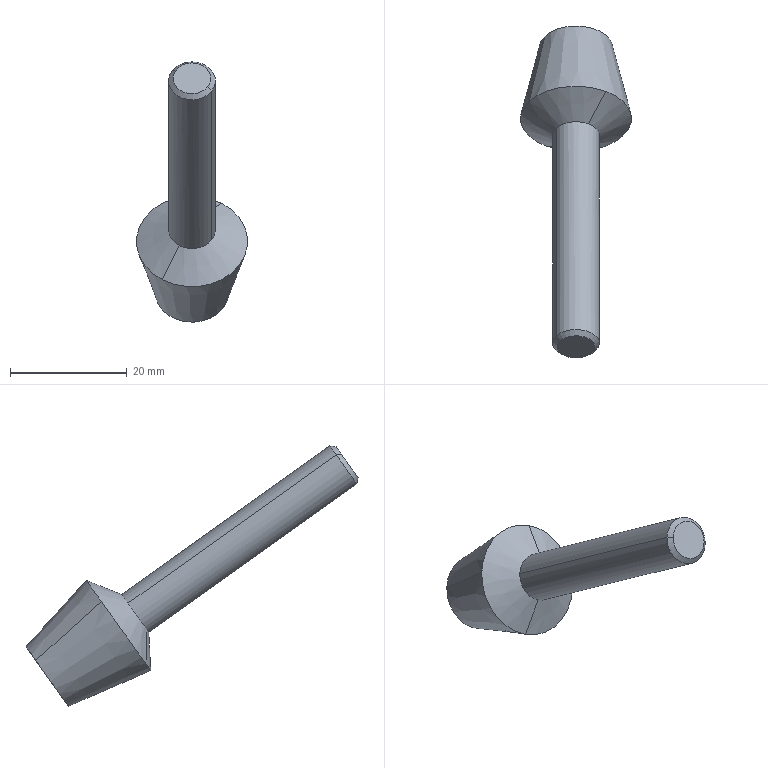Component | SolidWorks | AD12-MC01H-4_2_03.SDASM-1_AD12-_MC01H-4_bo.sdprt-1 | 1 solid | 10 faces | box 19 x 56.78 x 44.52 mm | volume 5722 mm3 | cone 6 | cylinder 2 | plane 2 | commonest cylinder face diameters 8 x2
STEP:
#1=COLOUR_RGB('',0.7922,0.8196,0.9333);
#2=FILL_AREA_STYLE_COLOUR('',#1);
#3=FILL_AREA_STYLE('',(#2));
#4=SURFACE_STYLE_FILL_AREA(#3);
#5=SURFACE_SIDE_STYLE('',(#4));
#6=SURFACE_STYLE_USAGE(.BOTH.,#5);
#7=PRESENTATION_STYLE_ASSIGNMENT((#6));
#8=CARTESIAN_POINT('',(-12.196,-6.944,14.752));
#9=VERTEX_POINT('',#8);
#10=CARTESIAN_POINT('',(-12.413,-6.972,14.713));
#11=VERTEX_POINT('',#10);
#12=CARTESIAN_POINT('',(-12.28,-7.021,14.644));
#13=DIRECTION('',(0.,-0.8137,0.5813));
#14=DIRECTION('',(0.8451,-0.3107,-0.435));
#15=AXIS2_PLACEMENT_3D('',#12,#13,#14);
#16=CIRCLE('',#15,0.1575);
#17=EDGE_CURVE('',#9,#11,#16,.T.);
#18=ORIENTED_EDGE('',*,*,#17,.T.);
#19=CARTESIAN_POINT('',(-12.413,-8.373,15.714));
#20=VERTEX_POINT('',#19);
#21=CARTESIAN_POINT('',(-12.413,-6.38,14.289));
#22=DIRECTION('',(0.,-0.8137,0.5813));
#23=VECTOR('',#22,39.37);
#24=LINE('',#21,#23);
#25=EDGE_CURVE('',#11,#20,#24,.T.);
#26=ORIENTED_EDGE('',*,*,#25,.T.);
#27=CARTESIAN_POINT('',(-12.147,-8.471,15.577));
#28=VERTEX_POINT('',#27);
#29=CARTESIAN_POINT('',(-12.28,-8.422,15.645));
#30=DIRECTION('',(-0.,0.8137,-0.5813));
#31=DIRECTION('',(0.8451,-0.3107,-0.435));
#32=AXIS2_PLACEMENT_3D('',#29,#30,#31);
#33=CIRCLE('',#32,0.1575);
#34=EDGE_CURVE('',#20,#28,#33,.T.);
#35=ORIENTED_EDGE('',*,*,#34,.T.);
#36=CARTESIAN_POINT('',(-12.147,-7.07,14.576));
#37=VERTEX_POINT('',#36);
#38=CARTESIAN_POINT('',(-12.147,-6.478,14.152));
#39=DIRECTION('',(0.,-0.8137,0.5813));
#40=VECTOR('',#39,39.37);
#41=LINE('',#38,#40);
#42=EDGE_CURVE('',#37,#28,#41,.T.);
#43=ORIENTED_EDGE('',*,*,#42,.F.);
#44=CARTESIAN_POINT('',(-12.28,-7.021,14.644));
#45=DIRECTION('',(0.,-0.8137,0.5813));
#46=DIRECTION('',(0.8451,-0.3107,-0.435));
#47=AXIS2_PLACEMENT_3D('',#44,#45,#46);
#48=CIRCLE('',#47,0.1575);
#49=EDGE_CURVE('',#37,#9,#48,.T.);
#50=ORIENTED_EDGE('',*,*,#49,.T.);
#51=EDGE_LOOP('',(#18,#26,#35,#43,#50));
#52=FACE_OUTER_BOUND('',#51,.T.);
#53=CARTESIAN_POINT('',(-12.28,-6.429,14.221));
#54=DIRECTION('',(0.,-0.8137,0.5813));
#55=DIRECTION('',(0.8451,-0.3107,-0.435));
#56=AXIS2_PLACEMENT_3D('',#53,#54,#55);
#57=CYLINDRICAL_SURFACE('',#56,0.1575);
#58=ADVANCED_FACE('',(#52),#57,.T.);
#59=CARTESIAN_POINT('',(-12.388,-8.407,15.718));
#60=VERTEX_POINT('',#59);
#61=CARTESIAN_POINT('',(-12.173,-8.486,15.607));
#62=VERTEX_POINT('',#61);
#63=CARTESIAN_POINT('',(-12.28,-8.447,15.663));
#64=DIRECTION('',(-0.,0.8137,-0.5813));
#65=DIRECTION('',(-0.8451,0.3107,0.435));
#66=AXIS2_PLACEMENT_3D('',#63,#64,#65);
#67=CIRCLE('',#66,0.1273);
#68=EDGE_CURVE('',#60,#62,#67,.T.);
#69=ORIENTED_EDGE('',*,*,#68,.T.);
#70=CARTESIAN_POINT('',(-12.147,-8.471,15.577));
#71=DIRECTION('',(0.5976,0.3556,-0.7186));
#72=VECTOR('',#71,39.37);
#73=LINE('',#70,#72);
#74=EDGE_CURVE('',#62,#28,#73,.T.);
#75=ORIENTED_EDGE('',*,*,#74,.T.);
#76=ORIENTED_EDGE('',*,*,#34,.F.);
#77=CARTESIAN_POINT('',(-12.413,-8.373,15.714));
#78=DIRECTION('',(-0.5976,0.7951,-0.1035));
#79=VECTOR('',#78,39.37);
#80=LINE('',#77,#79);
#81=EDGE_CURVE('',#60,#20,#80,.T.);
#82=ORIENTED_EDGE('',*,*,#81,.F.);
#83=EDGE_LOOP('',(#69,#75,#76,#82));
#84=FACE_OUTER_BOUND('',#83,.T.);
#85=CARTESIAN_POINT('',(-12.28,-8.422,15.645));
#86=DIRECTION('',(-0.,0.8137,-0.5813));
#87=DIRECTION('',(-0.8451,0.3107,0.435));
#88=AXIS2_PLACEMENT_3D('',#85,#86,#87);
#89=CONICAL_SURFACE('',#88,0.1575,0.7854);
#90=ADVANCED_FACE('',(#84),#89,.T.);
#91=CARTESIAN_POINT('',(-12.364,-7.099,14.536));
#92=VERTEX_POINT('',#91);
#93=CARTESIAN_POINT('',(-12.28,-7.021,14.644));
#94=DIRECTION('',(0.,-0.8137,0.5813));
#95=DIRECTION('',(0.8451,-0.3107,-0.435));
#96=AXIS2_PLACEMENT_3D('',#93,#94,#95);
#97=CIRCLE('',#96,0.1575);
#98=EDGE_CURVE('',#92,#37,#97,.T.);
#99=ORIENTED_EDGE('',*,*,#98,.F.);
#100=CARTESIAN_POINT('',(-12.48,-7.093,14.307));
#101=VERTEX_POINT('',#100);
#102=CARTESIAN_POINT('',(-12.48,-7.093,14.307));
#103=DIRECTION('',(-0.451,0.02239,-0.8922));
#104=VECTOR('',#103,39.37);
#105=LINE('',#102,#104);
#106=EDGE_CURVE('',#92,#101,#105,.T.);
#107=ORIENTED_EDGE('',*,*,#106,.T.);
#108=CARTESIAN_POINT('',(-11.964,-7.025,14.401));
#109=VERTEX_POINT('',#108);
#110=CARTESIAN_POINT('',(-12.28,-6.909,14.564));
#111=DIRECTION('',(0.,-0.8137,0.5813));
#112=DIRECTION('',(-0.8451,0.3107,0.435));
#113=AXIS2_PLACEMENT_3D('',#110,#111,#112);
#114=CIRCLE('',#113,0.374);
#115=EDGE_CURVE('',#101,#109,#114,.T.);
#116=ORIENTED_EDGE('',*,*,#115,.T.);
#117=CARTESIAN_POINT('',(-12.08,-6.725,14.821));
#118=VERTEX_POINT('',#117);
#119=CARTESIAN_POINT('',(-12.28,-6.909,14.564));
#120=DIRECTION('',(0.,-0.8137,0.5813));
#121=DIRECTION('',(-0.8451,0.3107,0.435));
#122=AXIS2_PLACEMENT_3D('',#119,#120,#121);
#123=CIRCLE('',#122,0.374);
#124=EDGE_CURVE('',#109,#118,#123,.T.);
#125=ORIENTED_EDGE('',*,*,#124,.T.);
#126=CARTESIAN_POINT('',(-12.08,-6.725,14.821));
#127=DIRECTION('',(0.451,0.8513,0.2681));
#128=VECTOR('',#127,39.37);
#129=LINE('',#126,#128);
#130=EDGE_CURVE('',#9,#118,#129,.T.);
#131=ORIENTED_EDGE('',*,*,#130,.F.);
#132=ORIENTED_EDGE('',*,*,#49,.F.);
#133=EDGE_LOOP('',(#99,#107,#116,#125,#131,#132));
#134=FACE_OUTER_BOUND('',#133,.T.);
#135=CARTESIAN_POINT('',(-12.28,-6.909,14.564));
#136=DIRECTION('',(0.,0.8137,-0.5813));
#137=DIRECTION('',(0.5346,0.4913,0.6877));
#138=AXIS2_PLACEMENT_3D('',#135,#136,#137);
#139=CONICAL_SURFACE('',#138,0.374,1.004);
#140=ADVANCED_FACE('',(#134),#139,.T.);
#141=CARTESIAN_POINT('',(-12.072,-6.505,14.114));
#142=VERTEX_POINT('',#141);
#143=CARTESIAN_POINT('',(-12.488,-6.352,14.328));
#144=VERTEX_POINT('',#143);
#145=CARTESIAN_POINT('',(-12.28,-6.429,14.221));
#146=DIRECTION('',(0.,-0.8137,0.5813));
#147=DIRECTION('',(0.8451,-0.3107,-0.435));
#148=AXIS2_PLACEMENT_3D('',#145,#146,#147);
#149=CIRCLE('',#148,0.2461);
#150=EDGE_CURVE('',#142,#144,#149,.T.);
#151=ORIENTED_EDGE('',*,*,#150,.T.);
#152=CARTESIAN_POINT('',(-12.596,-6.793,14.727));
#153=VERTEX_POINT('',#152);
#154=CARTESIAN_POINT('',(-12.596,-6.793,14.727));
#155=DIRECTION('',(-0.179,-0.7294,0.6602));
#156=VECTOR('',#155,39.37);
#157=LINE('',#154,#156);
#158=EDGE_CURVE('',#144,#153,#157,.T.);
#159=ORIENTED_EDGE('',*,*,#158,.T.);
#160=CARTESIAN_POINT('',(-12.28,-6.909,14.564));
#161=DIRECTION('',(0.,-0.8137,0.5813));
#162=DIRECTION('',(-0.8451,0.3107,0.435));
#163=AXIS2_PLACEMENT_3D('',#160,#161,#162);
#164=CIRCLE('',#163,0.374);
#165=EDGE_CURVE('',#118,#153,#164,.T.);
#166=ORIENTED_EDGE('',*,*,#165,.F.);
#167=ORIENTED_EDGE('',*,*,#124,.F.);
#168=CARTESIAN_POINT('',(-11.964,-7.025,14.401));
#169=DIRECTION('',(0.179,-0.861,0.476));
#170=VECTOR('',#169,39.37);
#171=LINE('',#168,#170);
#172=EDGE_CURVE('',#142,#109,#171,.T.);
#173=ORIENTED_EDGE('',*,*,#172,.F.);
#174=EDGE_LOOP('',(#151,#159,#166,#167,#173));
#175=FACE_OUTER_BOUND('',#174,.T.);
#176=CARTESIAN_POINT('',(-12.28,-6.909,14.564));
#177=DIRECTION('',(0.,-0.8137,0.5813));
#178=DIRECTION('',(0.8451,-0.3107,-0.435));
#179=AXIS2_PLACEMENT_3D('',#176,#177,#178);
#180=CONICAL_SURFACE('',#179,0.374,0.2134);
#181=ADVANCED_FACE('',(#175),#180,.T.);
#182=ORIENTED_EDGE('',*,*,#25,.F.);
#183=CARTESIAN_POINT('',(-12.28,-7.021,14.644));
#184=DIRECTION('',(0.,-0.8137,0.5813));
#185=DIRECTION('',(0.8451,-0.3107,-0.435));
#186=AXIS2_PLACEMENT_3D('',#183,#184,#185);
#187=CIRCLE('',#186,0.1575);
#188=EDGE_CURVE('',#11,#92,#187,.T.);
#189=ORIENTED_EDGE('',*,*,#188,.T.);
#190=ORIENTED_EDGE('',*,*,#98,.T.);
#191=ORIENTED_EDGE('',*,*,#42,.T.);
#192=CARTESIAN_POINT('',(-12.28,-8.422,15.645));
#193=DIRECTION('',(-0.,0.8137,-0.5813));
#194=DIRECTION('',(0.8451,-0.3107,-0.435));
#195=AXIS2_PLACEMENT_3D('',#192,#193,#194);
#196=CIRCLE('',#195,0.1575);
#197=EDGE_CURVE('',#28,#20,#196,.T.);
#198=ORIENTED_EDGE('',*,*,#197,.T.);
#199=EDGE_LOOP('',(#182,#189,#190,#191,#198));
#200=FACE_OUTER_BOUND('',#199,.T.);
#201=CARTESIAN_POINT('',(-12.28,-6.429,14.221));
#202=DIRECTION('',(0.,-0.8137,0.5813));
#203=DIRECTION('',(0.8451,-0.3107,-0.435));
#204=AXIS2_PLACEMENT_3D('',#201,#202,#203);
#205=CYLINDRICAL_SURFACE('',#204,0.1575);
#206=ADVANCED_FACE('',(#200),#205,.T.);
#207=ORIENTED_EDGE('',*,*,#74,.F.);
#208=CARTESIAN_POINT('',(-12.28,-8.447,15.663));
#209=DIRECTION('',(-0.,0.8137,-0.5813));
#210=DIRECTION('',(-0.8451,0.3107,0.435));
#211=AXIS2_PLACEMENT_3D('',#208,#209,#210);
#212=CIRCLE('',#211,0.1273);
#213=EDGE_CURVE('',#62,#60,#212,.T.);
#214=ORIENTED_EDGE('',*,*,#213,.T.);
#215=ORIENTED_EDGE('',*,*,#81,.T.);
#216=ORIENTED_EDGE('',*,*,#197,.F.);
#217=EDGE_LOOP('',(#207,#214,#215,#216));
#218=FACE_OUTER_BOUND('',#217,.T.);
#219=CARTESIAN_POINT('',(-12.28,-8.422,15.645));
#220=DIRECTION('',(-0.,0.8137,-0.5813));
#221=DIRECTION('',(-0.8451,0.3107,0.435));
#222=AXIS2_PLACEMENT_3D('',#219,#220,#221);
#223=CONICAL_SURFACE('',#222,0.1575,0.7854);
#224=ADVANCED_FACE('',(#218),#223,.T.);
#225=ORIENTED_EDGE('',*,*,#106,.F.);
#226=ORIENTED_EDGE('',*,*,#188,.F.);
#227=ORIENTED_EDGE('',*,*,#17,.F.);
#228=ORIENTED_EDGE('',*,*,#130,.T.);
#229=ORIENTED_EDGE('',*,*,#165,.T.);
#230=CARTESIAN_POINT('',(-12.28,-6.909,14.564));
#231=DIRECTION('',(0.,-0.8137,0.5813));
#232=DIRECTION('',(-0.8451,0.3107,0.435));
#233=AXIS2_PLACEMENT_3D('',#230,#231,#232);
#234=CIRCLE('',#233,0.374);
#235=EDGE_CURVE('',#153,#101,#234,.T.);
#236=ORIENTED_EDGE('',*,*,#235,.T.);
#237=EDGE_LOOP('',(#225,#226,#227,#228,#229,#236));
#238=FACE_OUTER_BOUND('',#237,.T.);
#239=CARTESIAN_POINT('',(-12.28,-6.909,14.564));
#240=DIRECTION('',(0.,0.8137,-0.5813));
#241=DIRECTION('',(0.5346,0.4913,0.6877));
#242=AXIS2_PLACEMENT_3D('',#239,#240,#241);
#243=CONICAL_SURFACE('',#242,0.374,1.004);
#244=ADVANCED_FACE('',(#238),#243,.T.);
#245=ORIENTED_EDGE('',*,*,#68,.F.);
#246=ORIENTED_EDGE('',*,*,#213,.F.);
#247=EDGE_LOOP('',(#245,#246));
#248=FACE_OUTER_BOUND('',#247,.T.);
#249=CARTESIAN_POINT('',(-12.28,-8.447,15.663));
#250=DIRECTION('',(0.,0.8137,-0.5813));
#251=DIRECTION('',(-0.8451,0.3107,0.435));
#252=AXIS2_PLACEMENT_3D('',#249,#250,#251);
#253=PLANE('',#252);
#254=ADVANCED_FACE('',(#248),#253,.F.);
#255=ORIENTED_EDGE('',*,*,#158,.F.);
#256=CARTESIAN_POINT('',(-12.28,-6.429,14.221));
#257=DIRECTION('',(0.,-0.8137,0.5813));
#258=DIRECTION('',(0.8451,-0.3107,-0.435));
#259=AXIS2_PLACEMENT_3D('',#256,#257,#258);
#260=CIRCLE('',#259,0.2461);
#261=EDGE_CURVE('',#144,#142,#260,.T.);
#262=ORIENTED_EDGE('',*,*,#261,.T.);
#263=ORIENTED_EDGE('',*,*,#172,.T.);
#264=ORIENTED_EDGE('',*,*,#115,.F.);
#265=ORIENTED_EDGE('',*,*,#235,.F.);
#266=EDGE_LOOP('',(#255,#262,#263,#264,#265));
#267=FACE_OUTER_BOUND('',#266,.T.);
#268=CARTESIAN_POINT('',(-12.28,-6.909,14.564));
#269=DIRECTION('',(0.,-0.8137,0.5813));
#270=DIRECTION('',(0.8451,-0.3107,-0.435));
#271=AXIS2_PLACEMENT_3D('',#268,#269,#270);
#272=CONICAL_SURFACE('',#271,0.374,0.2134);
#273=ADVANCED_FACE('',(#267),#272,.T.);
#274=ORIENTED_EDGE('',*,*,#150,.F.);
#275=ORIENTED_EDGE('',*,*,#261,.F.);
#276=EDGE_LOOP('',(#274,#275));
#277=FACE_OUTER_BOUND('',#276,.T.);
#278=CARTESIAN_POINT('',(-12.149,-6.308,14.39));
#279=DIRECTION('',(-0.,-0.8137,0.5813));
#280=DIRECTION('',(0.8451,-0.3107,-0.435));
#281=AXIS2_PLACEMENT_3D('',#278,#279,#280);
#282=PLANE('',#281);
#283=ADVANCED_FACE('',(#277),#282,.F.);
#284=CLOSED_SHELL('',(#58,#90,#140,#181,#206,#224,#244,#254,#273,#283));
#285=MANIFOLD_SOLID_BREP('',#284);
#286=STYLED_ITEM('',(#7),#285);
#287=PRESENTATION_LAYER_ASSIGNMENT('','',(#286));
#288=CARTESIAN_POINT('',(0.,0.,0.));
#289=DIRECTION('',(0.,0.,1.));
#290=DIRECTION('',(1.,0.,0.));
#291=AXIS2_PLACEMENT_3D('',#288,#289,#290);
#292=(LENGTH_UNIT()NAMED_UNIT(*)SI_UNIT($,.METRE.));
#293=LENGTH_MEASURE_WITH_UNIT(LENGTH_MEASURE(0.0254),#292);
#294=DIMENSIONAL_EXPONENTS(1.,0.,0.,0.,0.,0.,0.);
#295=(CONVERSION_BASED_UNIT('',#293)LENGTH_UNIT()NAMED_UNIT(#294));
#296=UNCERTAINTY_MEASURE_WITH_UNIT(LENGTH_MEASURE(0.00001),#295,'','');
#297=(NAMED_UNIT(*)PLANE_ANGLE_UNIT()SI_UNIT($,.RADIAN.));
#298=(NAMED_UNIT(*)SI_UNIT($,.STERADIAN.)SOLID_ANGLE_UNIT());
#299=(GEOMETRIC_REPRESENTATION_CONTEXT(3)GLOBAL_UNCERTAINTY_ASSIGNED_CONTEXT((#296))GLOBAL_UNIT_ASSIGNED_CONTEXT((#295,#297,#298))REPRESENTATION_CONTEXT('',''));
#300=ADVANCED_BREP_SHAPE_REPRESENTATION('',(#285,#291),#299);
#301=(LENGTH_UNIT()NAMED_UNIT(*)SI_UNIT($,.METRE.));
#302=LENGTH_MEASURE_WITH_UNIT(LENGTH_MEASURE(0.0254),#301);
#303=DIMENSIONAL_EXPONENTS(1.,0.,0.,0.,0.,0.,0.);
#304=(CONVERSION_BASED_UNIT('',#302)LENGTH_UNIT()NAMED_UNIT(#303));
#305=UNCERTAINTY_MEASURE_WITH_UNIT(LENGTH_MEASURE(0.00001),#304,'','');
#306=(NAMED_UNIT(*)PLANE_ANGLE_UNIT()SI_UNIT($,.RADIAN.));
#307=(NAMED_UNIT(*)SI_UNIT($,.STERADIAN.)SOLID_ANGLE_UNIT());
#308=(GEOMETRIC_REPRESENTATION_CONTEXT(3)GLOBAL_UNCERTAINTY_ASSIGNED_CONTEXT((#305))GLOBAL_UNIT_ASSIGNED_CONTEXT((#304,#306,#307))REPRESENTATION_CONTEXT('',''));
#309=MECHANICAL_DESIGN_GEOMETRIC_PRESENTATION_REPRESENTATION('',(#286),#308);